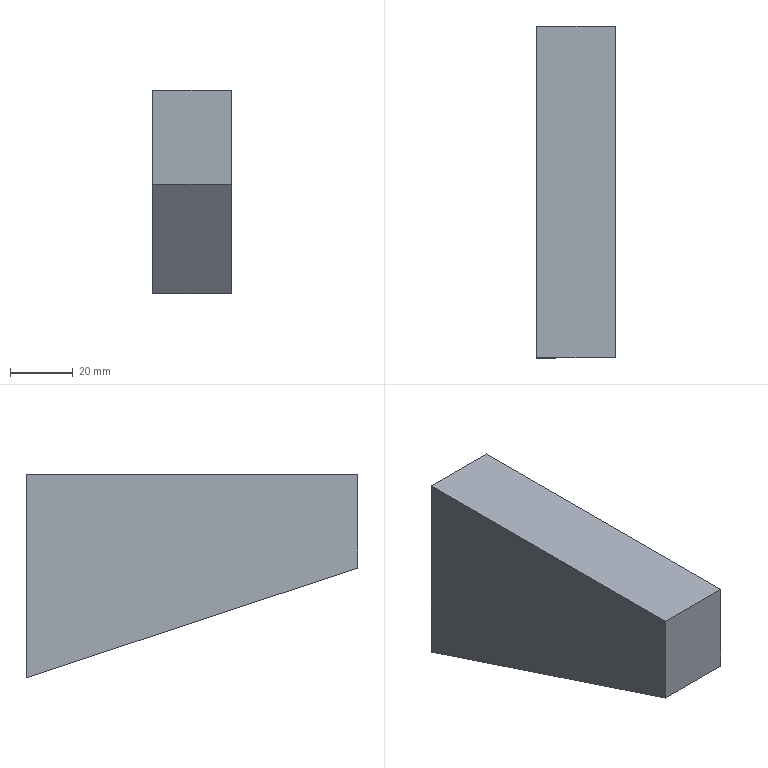Component | SolidWorks | MiddleHousing-1_Stiffener4-1 | 1 solid | 6 faces | box 25 x 106 x 65 mm | volume 125875 mm3 | plane 6
STEP:
#1=COLOUR_RGB('',0.7922,0.8196,0.9333);
#2=FILL_AREA_STYLE_COLOUR('',#1);
#3=FILL_AREA_STYLE('',(#2));
#4=SURFACE_STYLE_FILL_AREA(#3);
#5=SURFACE_SIDE_STYLE('',(#4));
#6=SURFACE_STYLE_USAGE(.BOTH.,#5);
#7=PRESENTATION_STYLE_ASSIGNMENT((#6));
#8=CARTESIAN_POINT('',(3.346,1.181,-7.48));
#9=VERTEX_POINT('',#8);
#10=CARTESIAN_POINT('',(3.346,5.354,-8.858));
#11=VERTEX_POINT('',#10);
#12=CARTESIAN_POINT('',(3.346,1.181,-7.48));
#13=DIRECTION('',(0.,0.9496,-0.3135));
#14=VECTOR('',#13,39.37);
#15=LINE('',#12,#14);
#16=EDGE_CURVE('',#9,#11,#15,.T.);
#17=ORIENTED_EDGE('',*,*,#16,.F.);
#18=CARTESIAN_POINT('',(3.346,1.181,-6.299));
#19=VERTEX_POINT('',#18);
#20=CARTESIAN_POINT('',(3.346,1.181,-8.858));
#21=DIRECTION('',(0.,0.,-1.));
#22=VECTOR('',#21,39.37);
#23=LINE('',#20,#22);
#24=EDGE_CURVE('',#19,#9,#23,.T.);
#25=ORIENTED_EDGE('',*,*,#24,.F.);
#26=CARTESIAN_POINT('',(3.346,5.354,-6.299));
#27=VERTEX_POINT('',#26);
#28=CARTESIAN_POINT('',(3.346,5.354,-6.299));
#29=DIRECTION('',(0.,-1.,0.));
#30=VECTOR('',#29,39.37);
#31=LINE('',#28,#30);
#32=EDGE_CURVE('',#27,#19,#31,.T.);
#33=ORIENTED_EDGE('',*,*,#32,.F.);
#34=CARTESIAN_POINT('',(3.346,5.354,-8.858));
#35=DIRECTION('',(0.,0.,1.));
#36=VECTOR('',#35,39.37);
#37=LINE('',#34,#36);
#38=EDGE_CURVE('',#11,#27,#37,.T.);
#39=ORIENTED_EDGE('',*,*,#38,.F.);
#40=EDGE_LOOP('',(#17,#25,#33,#39));
#41=FACE_OUTER_BOUND('',#40,.T.);
#42=CARTESIAN_POINT('',(3.346,5.354,-8.858));
#43=DIRECTION('',(1.,0.,0.));
#44=DIRECTION('',(0.,0.,-1.));
#45=AXIS2_PLACEMENT_3D('',#42,#43,#44);
#46=PLANE('',#45);
#47=ADVANCED_FACE('',(#41),#46,.F.);
#48=CARTESIAN_POINT('',(4.331,5.354,-8.858));
#49=VERTEX_POINT('',#48);
#50=CARTESIAN_POINT('',(4.331,5.354,-6.299));
#51=VERTEX_POINT('',#50);
#52=CARTESIAN_POINT('',(4.331,5.354,-8.858));
#53=DIRECTION('',(0.,0.,1.));
#54=VECTOR('',#53,39.37);
#55=LINE('',#52,#54);
#56=EDGE_CURVE('',#49,#51,#55,.T.);
#57=ORIENTED_EDGE('',*,*,#56,.F.);
#58=CARTESIAN_POINT('',(4.331,5.354,-8.858));
#59=DIRECTION('',(1.,0.,0.));
#60=VECTOR('',#59,39.37);
#61=LINE('',#58,#60);
#62=EDGE_CURVE('',#11,#49,#61,.T.);
#63=ORIENTED_EDGE('',*,*,#62,.F.);
#64=ORIENTED_EDGE('',*,*,#38,.T.);
#65=CARTESIAN_POINT('',(4.331,5.354,-6.299));
#66=DIRECTION('',(-1.,0.,0.));
#67=VECTOR('',#66,39.37);
#68=LINE('',#65,#67);
#69=EDGE_CURVE('',#51,#27,#68,.T.);
#70=ORIENTED_EDGE('',*,*,#69,.F.);
#71=EDGE_LOOP('',(#57,#63,#64,#70));
#72=FACE_OUTER_BOUND('',#71,.T.);
#73=CARTESIAN_POINT('',(4.331,5.354,-8.858));
#74=DIRECTION('',(0.,-1.,0.));
#75=DIRECTION('',(0.,0.,-1.));
#76=AXIS2_PLACEMENT_3D('',#73,#74,#75);
#77=PLANE('',#76);
#78=ADVANCED_FACE('',(#72),#77,.F.);
#79=ORIENTED_EDGE('',*,*,#16,.T.);
#80=ORIENTED_EDGE('',*,*,#62,.T.);
#81=CARTESIAN_POINT('',(4.331,1.181,-7.48));
#82=VERTEX_POINT('',#81);
#83=CARTESIAN_POINT('',(4.331,5.354,-8.858));
#84=DIRECTION('',(0.,0.9496,-0.3135));
#85=VECTOR('',#84,39.37);
#86=LINE('',#83,#85);
#87=EDGE_CURVE('',#82,#49,#86,.T.);
#88=ORIENTED_EDGE('',*,*,#87,.F.);
#89=CARTESIAN_POINT('',(-2.559,1.181,-7.48));
#90=DIRECTION('',(1.,0.,0.));
#91=VECTOR('',#90,39.37);
#92=LINE('',#89,#91);
#93=EDGE_CURVE('',#9,#82,#92,.T.);
#94=ORIENTED_EDGE('',*,*,#93,.F.);
#95=EDGE_LOOP('',(#79,#80,#88,#94));
#96=FACE_OUTER_BOUND('',#95,.T.);
#97=CARTESIAN_POINT('',(-2.559,5.354,-8.858));
#98=DIRECTION('',(0.,0.3135,0.9496));
#99=DIRECTION('',(0.,-0.9496,0.3135));
#100=AXIS2_PLACEMENT_3D('',#97,#98,#99);
#101=PLANE('',#100);
#102=ADVANCED_FACE('',(#96),#101,.F.);
#103=ORIENTED_EDGE('',*,*,#93,.T.);
#104=CARTESIAN_POINT('',(4.331,1.181,-6.299));
#105=VERTEX_POINT('',#104);
#106=CARTESIAN_POINT('',(4.331,1.181,-8.858));
#107=DIRECTION('',(0.,0.,-1.));
#108=VECTOR('',#107,39.37);
#109=LINE('',#106,#108);
#110=EDGE_CURVE('',#105,#82,#109,.T.);
#111=ORIENTED_EDGE('',*,*,#110,.F.);
#112=CARTESIAN_POINT('',(3.346,1.181,-6.299));
#113=DIRECTION('',(1.,0.,0.));
#114=VECTOR('',#113,39.37);
#115=LINE('',#112,#114);
#116=EDGE_CURVE('',#19,#105,#115,.T.);
#117=ORIENTED_EDGE('',*,*,#116,.F.);
#118=ORIENTED_EDGE('',*,*,#24,.T.);
#119=EDGE_LOOP('',(#103,#111,#117,#118));
#120=FACE_OUTER_BOUND('',#119,.T.);
#121=CARTESIAN_POINT('',(3.346,1.181,-8.858));
#122=DIRECTION('',(0.,1.,0.));
#123=DIRECTION('',(0.,0.,1.));
#124=AXIS2_PLACEMENT_3D('',#121,#122,#123);
#125=PLANE('',#124);
#126=ADVANCED_FACE('',(#120),#125,.F.);
#127=ORIENTED_EDGE('',*,*,#32,.T.);
#128=ORIENTED_EDGE('',*,*,#116,.T.);
#129=CARTESIAN_POINT('',(4.331,0.9843,-6.299));
#130=DIRECTION('',(0.,1.,0.));
#131=VECTOR('',#130,39.37);
#132=LINE('',#129,#131);
#133=EDGE_CURVE('',#105,#51,#132,.T.);
#134=ORIENTED_EDGE('',*,*,#133,.T.);
#135=ORIENTED_EDGE('',*,*,#69,.T.);
#136=EDGE_LOOP('',(#127,#128,#134,#135));
#137=FACE_OUTER_BOUND('',#136,.T.);
#138=CARTESIAN_POINT('',(8.268,0.9843,-6.299));
#139=DIRECTION('',(0.,0.,1.));
#140=DIRECTION('',(1.,0.,0.));
#141=AXIS2_PLACEMENT_3D('',#138,#139,#140);
#142=PLANE('',#141);
#143=ADVANCED_FACE('',(#137),#142,.T.);
#144=ORIENTED_EDGE('',*,*,#87,.T.);
#145=ORIENTED_EDGE('',*,*,#56,.T.);
#146=ORIENTED_EDGE('',*,*,#133,.F.);
#147=ORIENTED_EDGE('',*,*,#110,.T.);
#148=EDGE_LOOP('',(#144,#145,#146,#147));
#149=FACE_OUTER_BOUND('',#148,.T.);
#150=CARTESIAN_POINT('',(4.331,1.181,-8.858));
#151=DIRECTION('',(-1.,-0.,0.));
#152=DIRECTION('',(0.,-1.,0.));
#153=AXIS2_PLACEMENT_3D('',#150,#151,#152);
#154=PLANE('',#153);
#155=ADVANCED_FACE('',(#149),#154,.F.);
#156=CLOSED_SHELL('',(#47,#78,#102,#126,#143,#155));
#157=MANIFOLD_SOLID_BREP('',#156);
#158=STYLED_ITEM('',(#7),#157);
#159=(LENGTH_UNIT()NAMED_UNIT(*)SI_UNIT($,.METRE.));
#160=LENGTH_MEASURE_WITH_UNIT(LENGTH_MEASURE(0.0254),#159);
#161=DIMENSIONAL_EXPONENTS(1.,0.,0.,0.,0.,0.,0.);
#162=(CONVERSION_BASED_UNIT('',#160)LENGTH_UNIT()NAMED_UNIT(#161));
#163=UNCERTAINTY_MEASURE_WITH_UNIT(LENGTH_MEASURE(0.00001),#162,'','');
#164=(NAMED_UNIT(*)PLANE_ANGLE_UNIT()SI_UNIT($,.RADIAN.));
#165=(NAMED_UNIT(*)SI_UNIT($,.STERADIAN.)SOLID_ANGLE_UNIT());
#166=(GEOMETRIC_REPRESENTATION_CONTEXT(3)GLOBAL_UNCERTAINTY_ASSIGNED_CONTEXT((#163))GLOBAL_UNIT_ASSIGNED_CONTEXT((#162,#164,#165))REPRESENTATION_CONTEXT('',''));
#167=MECHANICAL_DESIGN_GEOMETRIC_PRESENTATION_REPRESENTATION('',(#158),#166);
#168=PRESENTATION_LAYER_ASSIGNMENT('','',(#158));
#169=CARTESIAN_POINT('',(0.,0.,0.));
#170=DIRECTION('',(0.,0.,1.));
#171=DIRECTION('',(1.,0.,0.));
#172=AXIS2_PLACEMENT_3D('',#169,#170,#171);
#173=(LENGTH_UNIT()NAMED_UNIT(*)SI_UNIT($,.METRE.));
#174=LENGTH_MEASURE_WITH_UNIT(LENGTH_MEASURE(0.0254),#173);
#175=DIMENSIONAL_EXPONENTS(1.,0.,0.,0.,0.,0.,0.);
#176=(CONVERSION_BASED_UNIT('',#174)LENGTH_UNIT()NAMED_UNIT(#175));
#177=UNCERTAINTY_MEASURE_WITH_UNIT(LENGTH_MEASURE(0.00001),#176,'','');
#178=(NAMED_UNIT(*)PLANE_ANGLE_UNIT()SI_UNIT($,.RADIAN.));
#179=(NAMED_UNIT(*)SI_UNIT($,.STERADIAN.)SOLID_ANGLE_UNIT());
#180=(GEOMETRIC_REPRESENTATION_CONTEXT(3)GLOBAL_UNCERTAINTY_ASSIGNED_CONTEXT((#177))GLOBAL_UNIT_ASSIGNED_CONTEXT((#176,#178,#179))REPRESENTATION_CONTEXT('',''));
#181=ADVANCED_BREP_SHAPE_REPRESENTATION('',(#157,#172),#180);